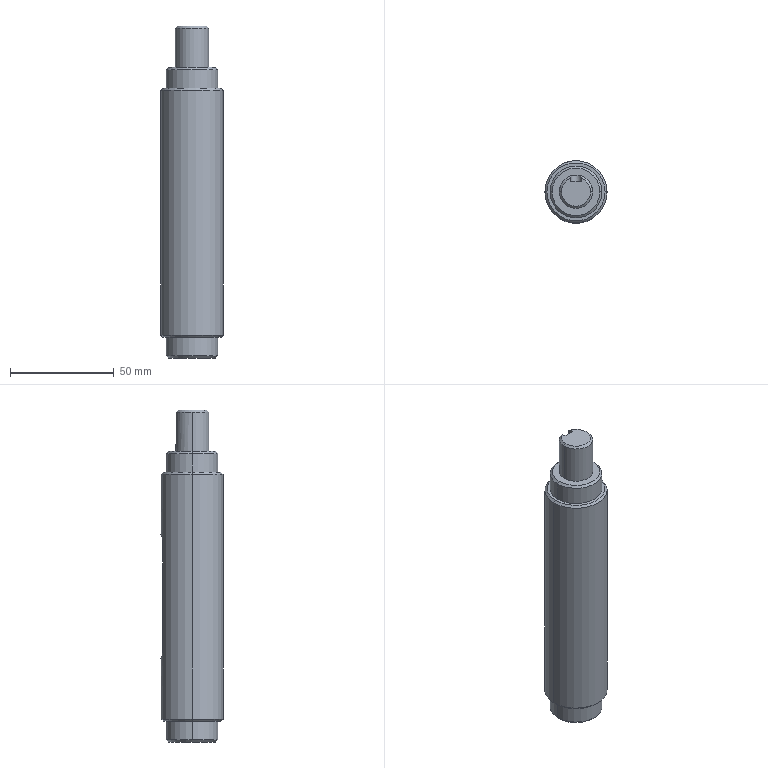Component | SolidWorks | WT-FLD-EJG-1212-00-008-1 | 1 solid | 33 faces | box 30 x 30 x 160 mm | volume 95493 mm3 | cone 11 | cylinder 11 | plane 11 | commonest cylinder face diameters 25 x4 30 x2 16 x2 10 x2 5 x1 | material AISI 1045 Steel, cold drawn
build123d program:
from build123d import *

# Parameters (mm, degrees)
CUT_EXTRUDE1_START  = 10
CUT_EXTRUDE1_DEPTH  = 64.144
SKETCH3_R           = 8
BOSS_EXTRUDE1_DEPTH = 20
CHAMFER1_SIZE       = 1
CUT_EXTRUDE2_START  = 5
CUT_EXTRUDE2_DEPTH  = 88.466


with BuildPart() as part:
    # Sketch1 → Revolve1 (revolve)
    with BuildSketch(Plane.XY, mode=Mode.PRIVATE) as revolve1_sk:
        Polygon((-70, 12.5), (-60, 12.5), (-60, 15), (60, 15), (60, 12.5), (70, 12.5), (70, 0), (-70, 0), align=None)
    revolve(revolve1_sk.sketch.rotate(Axis((-70, 0, 0), (1, 0, 0)), 90), axis=Axis((-70, 0, 0), (1, 0, 0)))

    # Sketch2 → Cut-Extrude1 (cut, through all)
    with BuildSketch(Plane(origin=(0, 0, 0), x_dir=(1, 0, 0), z_dir=(0, 1, 0)).offset(CUT_EXTRUDE1_START)):
        with BuildLine():
            Line((-25, 5), (25, 5))
            ThreePointArc((25, 5), (30, 0), (25, -5))
            Line((25, -5), (-25, -5))
            ThreePointArc((-25, -5), (-30, 0), (-25, 5))
        make_face()
    extrude(amount=CUT_EXTRUDE1_DEPTH, mode=Mode.SUBTRACT)

    # Sketch3 → Boss-Extrude1 (add)
    with BuildSketch(Plane(origin=(70, 0, 0), x_dir=(0, 0, -1), z_dir=(1, 0, 0))):
        with Locations(Location((0, 0, 0), (0, 0, 180))):
            Circle(SKETCH3_R)
    extrude(amount=BOSS_EXTRUDE1_DEPTH)

    # Chamfer1
    chamfer1_edges = [part.edges().sort_by_distance(p)[0] for p in [
        (90, 0, -8),
        (-70, 0, -12.5),
        (-60, 0, -15),
        (60, 0, -15),
        (70, 0, -12.5),
    ]]
    chamfer(chamfer1_edges, length=CHAMFER1_SIZE)

    # Sketch4 → Cut-Extrude2 (cut, through all)
    with BuildSketch(Plane(origin=(0, 0, 0), x_dir=(1, 0, 0), z_dir=(0, 1, 0)).offset(CUT_EXTRUDE2_START)):
        with BuildLine():
            Line((75, 2.5), (95, 2.5))
            ThreePointArc((95, 2.5), (97.5, 0), (95, -2.5))
            Line((95, -2.5), (75, -2.5))
            ThreePointArc((75, -2.5), (72.5, 0), (75, 2.5))
        make_face()
    extrude(amount=CUT_EXTRUDE2_DEPTH, mode=Mode.SUBTRACT)


solid = part.part

# Placed as in the assembly
solid = solid.moved(Location((0, 0, 0), (0, -90, 0)))
STEP:
#1=COLOUR_RGB('',0.7922,0.8196,0.9333);
#2=FILL_AREA_STYLE_COLOUR('',#1);
#3=FILL_AREA_STYLE('',(#2));
#4=SURFACE_STYLE_FILL_AREA(#3);
#5=SURFACE_SIDE_STYLE('',(#4));
#6=SURFACE_STYLE_USAGE(.BOTH.,#5);
#7=PRESENTATION_STYLE_ASSIGNMENT((#6));
#8=CARTESIAN_POINT('',(-0.5512,0.,-2.362));
#9=VERTEX_POINT('',#8);
#10=CARTESIAN_POINT('',(0.5512,0.,-2.362));
#11=VERTEX_POINT('',#10);
#12=CARTESIAN_POINT('',(0.,0.,-2.362));
#13=DIRECTION('',(0.,0.,-1.));
#14=DIRECTION('',(1.,0.,0.));
#15=AXIS2_PLACEMENT_3D('',#12,#13,#14);
#16=CIRCLE('',#15,0.5512);
#17=EDGE_CURVE('',#9,#11,#16,.T.);
#18=ORIENTED_EDGE('',*,*,#17,.F.);
#19=CARTESIAN_POINT('',(-0.5906,-0.,-2.323));
#20=VERTEX_POINT('',#19);
#21=CARTESIAN_POINT('',(-0.5512,0.,-2.362));
#22=DIRECTION('',(-0.7071,0.,0.7071));
#23=VECTOR('',#22,39.37);
#24=LINE('',#21,#23);
#25=EDGE_CURVE('',#9,#20,#24,.T.);
#26=ORIENTED_EDGE('',*,*,#25,.T.);
#27=CARTESIAN_POINT('',(0.5906,0.,-2.323));
#28=VERTEX_POINT('',#27);
#29=CARTESIAN_POINT('',(0.,0.,-2.323));
#30=DIRECTION('',(0.,0.,1.));
#31=DIRECTION('',(1.,0.,0.));
#32=AXIS2_PLACEMENT_3D('',#29,#30,#31);
#33=CIRCLE('',#32,0.5906);
#34=EDGE_CURVE('',#28,#20,#33,.T.);
#35=ORIENTED_EDGE('',*,*,#34,.F.);
#36=CARTESIAN_POINT('',(0.5512,0.,-2.362));
#37=DIRECTION('',(0.7071,0.,0.7071));
#38=VECTOR('',#37,39.37);
#39=LINE('',#36,#38);
#40=EDGE_CURVE('',#11,#28,#39,.T.);
#41=ORIENTED_EDGE('',*,*,#40,.F.);
#42=EDGE_LOOP('',(#18,#26,#35,#41));
#43=FACE_OUTER_BOUND('',#42,.T.);
#44=CARTESIAN_POINT('',(0.,0.,-2.362));
#45=DIRECTION('',(0.,0.,1.));
#46=DIRECTION('',(1.,0.,0.));
#47=AXIS2_PLACEMENT_3D('',#44,#45,#46);
#48=CONICAL_SURFACE('',#47,0.5512,0.7854);
#49=ADVANCED_FACE('',(#43),#48,.T.);
#50=CARTESIAN_POINT('',(-0.4528,0.,-2.756));
#51=VERTEX_POINT('',#50);
#52=CARTESIAN_POINT('',(0.4528,0.,-2.756));
#53=VERTEX_POINT('',#52);
#54=CARTESIAN_POINT('',(0.,0.,-2.756));
#55=DIRECTION('',(0.,0.,-1.));
#56=DIRECTION('',(1.,0.,0.));
#57=AXIS2_PLACEMENT_3D('',#54,#55,#56);
#58=CIRCLE('',#57,0.4528);
#59=EDGE_CURVE('',#51,#53,#58,.T.);
#60=ORIENTED_EDGE('',*,*,#59,.F.);
#61=CARTESIAN_POINT('',(-0.4921,-0.,-2.717));
#62=VERTEX_POINT('',#61);
#63=CARTESIAN_POINT('',(-0.4528,0.,-2.756));
#64=DIRECTION('',(-0.7071,0.,0.7071));
#65=VECTOR('',#64,39.37);
#66=LINE('',#63,#65);
#67=EDGE_CURVE('',#51,#62,#66,.T.);
#68=ORIENTED_EDGE('',*,*,#67,.T.);
#69=CARTESIAN_POINT('',(0.4921,0.,-2.717));
#70=VERTEX_POINT('',#69);
#71=CARTESIAN_POINT('',(0.,0.,-2.717));
#72=DIRECTION('',(0.,0.,1.));
#73=DIRECTION('',(1.,0.,0.));
#74=AXIS2_PLACEMENT_3D('',#71,#72,#73);
#75=CIRCLE('',#74,0.4921);
#76=EDGE_CURVE('',#70,#62,#75,.T.);
#77=ORIENTED_EDGE('',*,*,#76,.F.);
#78=CARTESIAN_POINT('',(0.4528,0.,-2.756));
#79=DIRECTION('',(0.7071,0.,0.7071));
#80=VECTOR('',#79,39.37);
#81=LINE('',#78,#80);
#82=EDGE_CURVE('',#53,#70,#81,.T.);
#83=ORIENTED_EDGE('',*,*,#82,.F.);
#84=EDGE_LOOP('',(#60,#68,#77,#83));
#85=FACE_OUTER_BOUND('',#84,.T.);
#86=CARTESIAN_POINT('',(0.,0.,-2.756));
#87=DIRECTION('',(0.,0.,1.));
#88=DIRECTION('',(1.,0.,0.));
#89=AXIS2_PLACEMENT_3D('',#86,#87,#88);
#90=CONICAL_SURFACE('',#89,0.4528,0.7854);
#91=ADVANCED_FACE('',(#85),#90,.T.);
#92=CARTESIAN_POINT('',(0.5512,0.,2.362));
#93=VERTEX_POINT('',#92);
#94=CARTESIAN_POINT('',(-0.5512,-0.,2.362));
#95=VERTEX_POINT('',#94);
#96=CARTESIAN_POINT('',(0.,0.,2.362));
#97=DIRECTION('',(0.,0.,1.));
#98=DIRECTION('',(-1.,-0.,0.));
#99=AXIS2_PLACEMENT_3D('',#96,#97,#98);
#100=CIRCLE('',#99,0.5512);
#101=EDGE_CURVE('',#93,#95,#100,.T.);
#102=ORIENTED_EDGE('',*,*,#101,.F.);
#103=CARTESIAN_POINT('',(0.5906,0.,2.323));
#104=VERTEX_POINT('',#103);
#105=CARTESIAN_POINT('',(0.5906,0.,2.323));
#106=DIRECTION('',(0.7071,0.,-0.7071));
#107=VECTOR('',#106,39.37);
#108=LINE('',#105,#107);
#109=EDGE_CURVE('',#93,#104,#108,.T.);
#110=ORIENTED_EDGE('',*,*,#109,.T.);
#111=CARTESIAN_POINT('',(-0.5906,-0.,2.323));
#112=VERTEX_POINT('',#111);
#113=CARTESIAN_POINT('',(0.,0.,2.323));
#114=DIRECTION('',(0.,0.,-1.));
#115=DIRECTION('',(-1.,-0.,0.));
#116=AXIS2_PLACEMENT_3D('',#113,#114,#115);
#117=CIRCLE('',#116,0.5906);
#118=EDGE_CURVE('',#112,#104,#117,.T.);
#119=ORIENTED_EDGE('',*,*,#118,.F.);
#120=CARTESIAN_POINT('',(-0.5906,-0.,2.323));
#121=DIRECTION('',(-0.7071,-0.,-0.7071));
#122=VECTOR('',#121,39.37);
#123=LINE('',#120,#122);
#124=EDGE_CURVE('',#95,#112,#123,.T.);
#125=ORIENTED_EDGE('',*,*,#124,.F.);
#126=EDGE_LOOP('',(#102,#110,#119,#125));
#127=FACE_OUTER_BOUND('',#126,.T.);
#128=CARTESIAN_POINT('',(0.,0.,2.323));
#129=DIRECTION('',(0.,0.,-1.));
#130=DIRECTION('',(-1.,-0.,0.));
#131=AXIS2_PLACEMENT_3D('',#128,#129,#130);
#132=CONICAL_SURFACE('',#131,0.5906,0.7854);
#133=ADVANCED_FACE('',(#127),#132,.T.);
#134=CARTESIAN_POINT('',(0.4528,0.,2.756));
#135=VERTEX_POINT('',#134);
#136=CARTESIAN_POINT('',(-0.4528,-0.,2.756));
#137=VERTEX_POINT('',#136);
#138=CARTESIAN_POINT('',(0.,0.,2.756));
#139=DIRECTION('',(0.,0.,1.));
#140=DIRECTION('',(-1.,-0.,0.));
#141=AXIS2_PLACEMENT_3D('',#138,#139,#140);
#142=CIRCLE('',#141,0.4528);
#143=EDGE_CURVE('',#135,#137,#142,.T.);
#144=ORIENTED_EDGE('',*,*,#143,.F.);
#145=CARTESIAN_POINT('',(0.4921,0.,2.717));
#146=VERTEX_POINT('',#145);
#147=CARTESIAN_POINT('',(0.4921,0.,2.717));
#148=DIRECTION('',(0.7071,0.,-0.7071));
#149=VECTOR('',#148,39.37);
#150=LINE('',#147,#149);
#151=EDGE_CURVE('',#135,#146,#150,.T.);
#152=ORIENTED_EDGE('',*,*,#151,.T.);
#153=CARTESIAN_POINT('',(-0.4921,-0.,2.717));
#154=VERTEX_POINT('',#153);
#155=CARTESIAN_POINT('',(0.,0.,2.717));
#156=DIRECTION('',(0.,0.,-1.));
#157=DIRECTION('',(-1.,-0.,0.));
#158=AXIS2_PLACEMENT_3D('',#155,#156,#157);
#159=CIRCLE('',#158,0.4921);
#160=EDGE_CURVE('',#154,#146,#159,.T.);
#161=ORIENTED_EDGE('',*,*,#160,.F.);
#162=CARTESIAN_POINT('',(-0.4921,-0.,2.717));
#163=DIRECTION('',(-0.7071,-0.,-0.7071));
#164=VECTOR('',#163,39.37);
#165=LINE('',#162,#164);
#166=EDGE_CURVE('',#137,#154,#165,.T.);
#167=ORIENTED_EDGE('',*,*,#166,.F.);
#168=EDGE_LOOP('',(#144,#152,#161,#167));
#169=FACE_OUTER_BOUND('',#168,.T.);
#170=CARTESIAN_POINT('',(0.,0.,2.717));
#171=DIRECTION('',(0.,0.,-1.));
#172=DIRECTION('',(-1.,-0.,0.));
#173=AXIS2_PLACEMENT_3D('',#170,#171,#172);
#174=CONICAL_SURFACE('',#173,0.4921,0.7854);
#175=ADVANCED_FACE('',(#169),#174,.T.);
#176=CARTESIAN_POINT('',(-0.4921,-0.,-2.362));
#177=VERTEX_POINT('',#176);
#178=CARTESIAN_POINT('',(0.4921,0.,-2.362));
#179=VERTEX_POINT('',#178);
#180=CARTESIAN_POINT('',(0.,0.,-2.362));
#181=DIRECTION('',(0.,0.,-1.));
#182=DIRECTION('',(-1.,-0.,0.));
#183=AXIS2_PLACEMENT_3D('',#180,#181,#182);
#184=CIRCLE('',#183,0.4921);
#185=EDGE_CURVE('',#177,#179,#184,.T.);
#186=ORIENTED_EDGE('',*,*,#185,.T.);
#187=CARTESIAN_POINT('',(0.4921,0.,-2.756));
#188=DIRECTION('',(0.,0.,-1.));
#189=VECTOR('',#188,39.37);
#190=LINE('',#187,#189);
#191=EDGE_CURVE('',#179,#70,#190,.T.);
#192=ORIENTED_EDGE('',*,*,#191,.T.);
#193=ORIENTED_EDGE('',*,*,#76,.T.);
#194=CARTESIAN_POINT('',(-0.4921,-0.,-2.756));
#195=DIRECTION('',(0.,0.,-1.));
#196=VECTOR('',#195,39.37);
#197=LINE('',#194,#196);
#198=EDGE_CURVE('',#177,#62,#197,.T.);
#199=ORIENTED_EDGE('',*,*,#198,.F.);
#200=EDGE_LOOP('',(#186,#192,#193,#199));
#201=FACE_OUTER_BOUND('',#200,.T.);
#202=CARTESIAN_POINT('',(0.,0.,-2.756));
#203=DIRECTION('',(0.,0.,-1.));
#204=DIRECTION('',(-1.,-0.,0.));
#205=AXIS2_PLACEMENT_3D('',#202,#203,#204);
#206=CYLINDRICAL_SURFACE('',#205,0.4921);
#207=ADVANCED_FACE('',(#201),#206,.T.);
#208=ORIENTED_EDGE('',*,*,#160,.T.);
#209=CARTESIAN_POINT('',(0.4921,0.,2.362));
#210=VERTEX_POINT('',#209);
#211=CARTESIAN_POINT('',(0.4921,0.,-2.756));
#212=DIRECTION('',(0.,0.,-1.));
#213=VECTOR('',#212,39.37);
#214=LINE('',#211,#213);
#215=EDGE_CURVE('',#146,#210,#214,.T.);
#216=ORIENTED_EDGE('',*,*,#215,.T.);
#217=CARTESIAN_POINT('',(-0.4921,-0.,2.362));
#218=VERTEX_POINT('',#217);
#219=CARTESIAN_POINT('',(0.,0.,2.362));
#220=DIRECTION('',(0.,0.,-1.));
#221=DIRECTION('',(-1.,-0.,0.));
#222=AXIS2_PLACEMENT_3D('',#219,#220,#221);
#223=CIRCLE('',#222,0.4921);
#224=EDGE_CURVE('',#218,#210,#223,.T.);
#225=ORIENTED_EDGE('',*,*,#224,.F.);
#226=CARTESIAN_POINT('',(-0.4921,-0.,-2.756));
#227=DIRECTION('',(0.,0.,-1.));
#228=VECTOR('',#227,39.37);
#229=LINE('',#226,#228);
#230=EDGE_CURVE('',#154,#218,#229,.T.);
#231=ORIENTED_EDGE('',*,*,#230,.F.);
#232=EDGE_LOOP('',(#208,#216,#225,#231));
#233=FACE_OUTER_BOUND('',#232,.T.);
#234=CARTESIAN_POINT('',(0.,0.,-2.756));
#235=DIRECTION('',(0.,0.,-1.));
#236=DIRECTION('',(-1.,-0.,0.));
#237=AXIS2_PLACEMENT_3D('',#234,#235,#236);
#238=CYLINDRICAL_SURFACE('',#237,0.4921);
#239=ADVANCED_FACE('',(#233),#238,.T.);
#240=CARTESIAN_POINT('',(-0.1969,0.5568,0.9843));
#241=VERTEX_POINT('',#240);
#242=CARTESIAN_POINT('',(0.1969,0.5568,0.9843));
#243=VERTEX_POINT('',#242);
#244=CARTESIAN_POINT('',(-0.1969,0.5568,0.9843));
#245=CARTESIAN_POINT('',(-0.1969,0.5568,0.9974));
#246=CARTESIAN_POINT('',(-0.1956,0.5572,1.01));
#247=CARTESIAN_POINT('',(-0.1905,0.559,1.035));
#248=CARTESIAN_POINT('',(-0.1867,0.5603,1.048));
#249=CARTESIAN_POINT('',(-0.1768,0.5635,1.072));
#250=CARTESIAN_POINT('',(-0.1707,0.5654,1.083));
#251=CARTESIAN_POINT('',(-0.1565,0.5695,1.104));
#252=CARTESIAN_POINT('',(-0.1482,0.5717,1.114));
#253=CARTESIAN_POINT('',(-0.1302,0.5761,1.132));
#254=CARTESIAN_POINT('',(-0.1204,0.5783,1.141));
#255=CARTESIAN_POINT('',(-0.09888,0.5823,1.155));
#256=CARTESIAN_POINT('',(-0.08758,0.5841,1.161));
#257=CARTESIAN_POINT('',(-0.06985,0.5864,1.168));
#258=CARTESIAN_POINT('',(-0.0638,0.5871,1.171));
#259=CARTESIAN_POINT('',(-0.05143,0.5883,1.174));
#260=CARTESIAN_POINT('',(-0.04507,0.5889,1.176));
#261=CARTESIAN_POINT('',(-0.02599,0.5901,1.18));
#262=CARTESIAN_POINT('',(-0.01315,0.5905,1.181));
#263=CARTESIAN_POINT('',(0.01273,0.5906,1.181));
#264=CARTESIAN_POINT('',(0.02588,0.5901,1.18));
#265=CARTESIAN_POINT('',(0.05121,0.5885,1.175));
#266=CARTESIAN_POINT('',(0.06353,0.5872,1.171));
#267=CARTESIAN_POINT('',(0.08749,0.5842,1.161));
#268=CARTESIAN_POINT('',(0.09885,0.5823,1.155));
#269=CARTESIAN_POINT('',(0.1201,0.5783,1.141));
#270=CARTESIAN_POINT('',(0.1301,0.5761,1.133));
#271=CARTESIAN_POINT('',(0.1482,0.5717,1.114));
#272=CARTESIAN_POINT('',(0.1563,0.5695,1.105));
#273=CARTESIAN_POINT('',(0.1706,0.5654,1.083));
#274=CARTESIAN_POINT('',(0.1768,0.5635,1.072));
#275=CARTESIAN_POINT('',(0.1866,0.5603,1.048));
#276=CARTESIAN_POINT('',(0.1904,0.559,1.036));
#277=CARTESIAN_POINT('',(0.1955,0.5572,1.01));
#278=CARTESIAN_POINT('',(0.1969,0.5568,0.9974));
#279=CARTESIAN_POINT('',(0.1969,0.5568,0.9843));
#280=B_SPLINE_CURVE_WITH_KNOTS('',3,(#244,#245,#246,#247,#248,#249,#250,#251,#252,#253,#254,#255,#256,#257,#258,#259,#260,#261,#262,#263,#264,#265,#266,#267,#268,#269,#270,#271,#272,#273,#274,#275,#276,#277,#278,#279),.UNSPECIFIED.,.F.,.F.,(4,2,2,2,2,2,2,2,2,2,2,2,2,2,2,2,2,4),(0.,0.0009837,0.001967,0.002951,0.003935,0.004919,0.005902,0.006394,0.006886,0.00787,0.008853,0.009837,0.01082,0.0118,0.01279,0.01377,0.01476,0.01574),.UNSPECIFIED.);
#281=EDGE_CURVE('',#241,#243,#280,.T.);
#282=ORIENTED_EDGE('',*,*,#281,.F.);
#283=CARTESIAN_POINT('',(-0.1969,0.5568,-0.9843));
#284=VERTEX_POINT('',#283);
#285=CARTESIAN_POINT('',(-0.1969,0.5568,-2.756));
#286=DIRECTION('',(0.,0.,1.));
#287=VECTOR('',#286,39.37);
#288=LINE('',#285,#287);
#289=EDGE_CURVE('',#284,#241,#288,.T.);
#290=ORIENTED_EDGE('',*,*,#289,.F.);
#291=CARTESIAN_POINT('',(0.1969,0.5568,-0.9843));
#292=VERTEX_POINT('',#291);
#293=CARTESIAN_POINT('',(0.1969,0.5568,-0.9843));
#294=CARTESIAN_POINT('',(0.1969,0.5568,-0.9974));
#295=CARTESIAN_POINT('',(0.1956,0.5572,-1.01));
#296=CARTESIAN_POINT('',(0.1905,0.559,-1.035));
#297=CARTESIAN_POINT('',(0.1867,0.5603,-1.048));
#298=CARTESIAN_POINT('',(0.1768,0.5635,-1.072));
#299=CARTESIAN_POINT('',(0.1707,0.5654,-1.083));
#300=CARTESIAN_POINT('',(0.1565,0.5695,-1.104));
#301=CARTESIAN_POINT('',(0.1482,0.5717,-1.114));
#302=CARTESIAN_POINT('',(0.1302,0.5761,-1.132));
#303=CARTESIAN_POINT('',(0.1204,0.5783,-1.141));
#304=CARTESIAN_POINT('',(0.09888,0.5823,-1.155));
#305=CARTESIAN_POINT('',(0.08758,0.5841,-1.161));
#306=CARTESIAN_POINT('',(0.06985,0.5864,-1.168));
#307=CARTESIAN_POINT('',(0.0638,0.5871,-1.171));
#308=CARTESIAN_POINT('',(0.05143,0.5883,-1.174));
#309=CARTESIAN_POINT('',(0.04507,0.5889,-1.176));
#310=CARTESIAN_POINT('',(0.02599,0.5901,-1.18));
#311=CARTESIAN_POINT('',(0.01315,0.5905,-1.181));
#312=CARTESIAN_POINT('',(-0.01273,0.5906,-1.181));
#313=CARTESIAN_POINT('',(-0.02588,0.5901,-1.18));
#314=CARTESIAN_POINT('',(-0.05121,0.5885,-1.175));
#315=CARTESIAN_POINT('',(-0.06353,0.5872,-1.171));
#316=CARTESIAN_POINT('',(-0.08749,0.5842,-1.161));
#317=CARTESIAN_POINT('',(-0.09885,0.5823,-1.155));
#318=CARTESIAN_POINT('',(-0.1201,0.5783,-1.141));
#319=CARTESIAN_POINT('',(-0.1301,0.5761,-1.133));
#320=CARTESIAN_POINT('',(-0.1482,0.5717,-1.114));
#321=CARTESIAN_POINT('',(-0.1563,0.5695,-1.105));
#322=CARTESIAN_POINT('',(-0.1706,0.5654,-1.083));
#323=CARTESIAN_POINT('',(-0.1768,0.5635,-1.072));
#324=CARTESIAN_POINT('',(-0.1866,0.5603,-1.048));
#325=CARTESIAN_POINT('',(-0.1904,0.559,-1.036));
#326=CARTESIAN_POINT('',(-0.1955,0.5572,-1.01));
#327=CARTESIAN_POINT('',(-0.1969,0.5568,-0.9974));
#328=CARTESIAN_POINT('',(-0.1969,0.5568,-0.9843));
#329=B_SPLINE_CURVE_WITH_KNOTS('',3,(#293,#294,#295,#296,#297,#298,#299,#300,#301,#302,#303,#304,#305,#306,#307,#308,#309,#310,#311,#312,#313,#314,#315,#316,#317,#318,#319,#320,#321,#322,#323,#324,#325,#326,#327,#328),.UNSPECIFIED.,.F.,.F.,(4,2,2,2,2,2,2,2,2,2,2,2,2,2,2,2,2,4),(0.,0.0009837,0.001967,0.002951,0.003935,0.004919,0.005902,0.006394,0.006886,0.00787,0.008853,0.009837,0.01082,0.0118,0.01279,0.01377,0.01476,0.01574),.UNSPECIFIED.);
#330=EDGE_CURVE('',#292,#284,#329,.T.);
#331=ORIENTED_EDGE('',*,*,#330,.F.);
#332=CARTESIAN_POINT('',(0.1969,0.5568,-2.756));
#333=DIRECTION('',(0.,0.,-1.));
#334=VECTOR('',#333,39.37);
#335=LINE('',#332,#334);
#336=EDGE_CURVE('',#243,#292,#335,.T.);
#337=ORIENTED_EDGE('',*,*,#336,.F.);
#338=EDGE_LOOP('',(#282,#290,#331,#337));
#339=FACE_BOUND('',#338,.T.);
#340=ORIENTED_EDGE('',*,*,#118,.T.);
#341=CARTESIAN_POINT('',(0.5906,0.,-2.756));
#342=DIRECTION('',(0.,0.,-1.));
#343=VECTOR('',#342,39.37);
#344=LINE('',#341,#343);
#345=EDGE_CURVE('',#104,#28,#344,.T.);
#346=ORIENTED_EDGE('',*,*,#345,.T.);
#347=ORIENTED_EDGE('',*,*,#34,.T.);
#348=CARTESIAN_POINT('',(-0.5906,-0.,-2.756));
#349=DIRECTION('',(0.,0.,-1.));
#350=VECTOR('',#349,39.37);
#351=LINE('',#348,#350);
#352=EDGE_CURVE('',#112,#20,#351,.T.);
#353=ORIENTED_EDGE('',*,*,#352,.F.);
#354=EDGE_LOOP('',(#340,#346,#347,#353));
#355=FACE_OUTER_BOUND('',#354,.T.);
#356=CARTESIAN_POINT('',(0.,0.,-2.756));
#357=DIRECTION('',(0.,0.,-1.));
#358=DIRECTION('',(-1.,-0.,0.));
#359=AXIS2_PLACEMENT_3D('',#356,#357,#358);
#360=CYLINDRICAL_SURFACE('',#359,0.5906);
#361=ADVANCED_FACE('',(#339,#355),#360,.T.);
#362=CARTESIAN_POINT('',(0.2756,0.,3.543));
#363=VERTEX_POINT('',#362);
#364=CARTESIAN_POINT('',(0.09843,0.2574,3.543));
#365=VERTEX_POINT('',#364);
#366=CARTESIAN_POINT('',(0.,0.,3.543));
#367=DIRECTION('',(0.,0.,1.));
#368=DIRECTION('',(1.,0.,0.));
#369=AXIS2_PLACEMENT_3D('',#366,#367,#368);
#370=CIRCLE('',#369,0.2756);
#371=EDGE_CURVE('',#363,#365,#370,.T.);
#372=ORIENTED_EDGE('',*,*,#371,.F.);
#373=CARTESIAN_POINT('',(0.315,0.,3.504));
#374=VERTEX_POINT('',#373);
#375=CARTESIAN_POINT('',(0.2756,0.,3.543));
#376=DIRECTION('',(0.7071,0.,-0.7071));
#377=VECTOR('',#376,39.37);
#378=LINE('',#375,#377);
#379=EDGE_CURVE('',#363,#374,#378,.T.);
#380=ORIENTED_EDGE('',*,*,#379,.T.);
#381=CARTESIAN_POINT('',(0.09843,0.2992,3.504));
#382=VERTEX_POINT('',#381);
#383=CARTESIAN_POINT('',(0.,0.,3.504));
#384=DIRECTION('',(0.,0.,-1.));
#385=DIRECTION('',(1.,-0.,0.));
#386=AXIS2_PLACEMENT_3D('',#383,#384,#385);
#387=CIRCLE('',#386,0.315);
#388=EDGE_CURVE('',#382,#374,#387,.T.);
#389=ORIENTED_EDGE('',*,*,#388,.F.);
#390=CARTESIAN_POINT('',(0.09843,0.2992,3.504));
#391=CARTESIAN_POINT('',(0.09843,0.2853,3.517));
#392=CARTESIAN_POINT('',(0.09843,0.2714,3.53));
#393=CARTESIAN_POINT('',(0.09843,0.2574,3.543));
#394=B_SPLINE_CURVE_WITH_KNOTS('',3,(#390,#391,#392,#393),.UNSPECIFIED.,.F.,.F.,(4,4),(0.005308,0.006766),.UNSPECIFIED.);
#395=EDGE_CURVE('',#382,#365,#394,.T.);
#396=ORIENTED_EDGE('',*,*,#395,.T.);
#397=EDGE_LOOP('',(#372,#380,#389,#396));
#398=FACE_OUTER_BOUND('',#397,.T.);
#399=CARTESIAN_POINT('',(0.,0.,3.543));
#400=DIRECTION('',(0.,0.,-1.));
#401=DIRECTION('',(-1.,-0.,0.));
#402=AXIS2_PLACEMENT_3D('',#399,#400,#401);
#403=CONICAL_SURFACE('',#402,0.2756,0.7854);
#404=ADVANCED_FACE('',(#398),#403,.T.);
#405=ORIENTED_EDGE('',*,*,#379,.F.);
#406=CARTESIAN_POINT('',(-0.2756,-0.,3.543));
#407=VERTEX_POINT('',#406);
#408=CARTESIAN_POINT('',(0.,0.,3.543));
#409=DIRECTION('',(0.,0.,1.));
#410=DIRECTION('',(1.,0.,0.));
#411=AXIS2_PLACEMENT_3D('',#408,#409,#410);
#412=CIRCLE('',#411,0.2756);
#413=EDGE_CURVE('',#407,#363,#412,.T.);
#414=ORIENTED_EDGE('',*,*,#413,.F.);
#415=CARTESIAN_POINT('',(-0.315,-0.,3.504));
#416=VERTEX_POINT('',#415);
#417=CARTESIAN_POINT('',(-0.2756,-0.,3.543));
#418=DIRECTION('',(-0.7071,-0.,-0.7071));
#419=VECTOR('',#418,39.37);
#420=LINE('',#417,#419);
#421=EDGE_CURVE('',#407,#416,#420,.T.);
#422=ORIENTED_EDGE('',*,*,#421,.T.);
#423=CARTESIAN_POINT('',(0.,0.,3.504));
#424=DIRECTION('',(0.,0.,-1.));
#425=DIRECTION('',(1.,0.,0.));
#426=AXIS2_PLACEMENT_3D('',#423,#424,#425);
#427=CIRCLE('',#426,0.315);
#428=EDGE_CURVE('',#374,#416,#427,.T.);
#429=ORIENTED_EDGE('',*,*,#428,.F.);
#430=EDGE_LOOP('',(#405,#414,#422,#429));
#431=FACE_OUTER_BOUND('',#430,.T.);
#432=CARTESIAN_POINT('',(0.,0.,3.543));
#433=DIRECTION('',(0.,0.,-1.));
#434=DIRECTION('',(-1.,-0.,0.));
#435=AXIS2_PLACEMENT_3D('',#432,#433,#434);
#436=CONICAL_SURFACE('',#435,0.2756,0.7854);
#437=ADVANCED_FACE('',(#431),#436,.T.);
#438=ORIENTED_EDGE('',*,*,#388,.T.);
#439=CARTESIAN_POINT('',(0.315,0.,2.756));
#440=VERTEX_POINT('',#439);
#441=CARTESIAN_POINT('',(0.315,0.,3.543));
#442=DIRECTION('',(0.,0.,-1.));
#443=VECTOR('',#442,39.37);
#444=LINE('',#441,#443);
#445=EDGE_CURVE('',#374,#440,#444,.T.);
#446=ORIENTED_EDGE('',*,*,#445,.T.);
#447=CARTESIAN_POINT('',(-0.315,-0.,2.756));
#448=VERTEX_POINT('',#447);
#449=CARTESIAN_POINT('',(0.,0.,2.756));
#450=DIRECTION('',(0.,0.,1.));
#451=DIRECTION('',(-1.,-0.,0.));
#452=AXIS2_PLACEMENT_3D('',#449,#450,#451);
#453=CIRCLE('',#452,0.315);
#454=EDGE_CURVE('',#440,#448,#453,.T.);
#455=ORIENTED_EDGE('',*,*,#454,.T.);
#456=CARTESIAN_POINT('',(-0.315,-0.,3.543));
#457=DIRECTION('',(0.,0.,-1.));
#458=VECTOR('',#457,39.37);
#459=LINE('',#456,#458);
#460=EDGE_CURVE('',#416,#448,#459,.T.);
#461=ORIENTED_EDGE('',*,*,#460,.F.);
#462=CARTESIAN_POINT('',(-0.09843,0.2992,3.504));
#463=VERTEX_POINT('',#462);
#464=CARTESIAN_POINT('',(0.,0.,3.504));
#465=DIRECTION('',(0.,0.,-1.));
#466=DIRECTION('',(1.,0.,0.));
#467=AXIS2_PLACEMENT_3D('',#464,#465,#466);
#468=CIRCLE('',#467,0.315);
#469=EDGE_CURVE('',#416,#463,#468,.T.);
#470=ORIENTED_EDGE('',*,*,#469,.T.);
#471=CARTESIAN_POINT('',(-0.09843,0.2992,2.953));
#472=VERTEX_POINT('',#471);
#473=CARTESIAN_POINT('',(-0.09843,0.2992,3.543));
#474=DIRECTION('',(0.,0.,1.));
#475=VECTOR('',#474,39.37);
#476=LINE('',#473,#475);
#477=EDGE_CURVE('',#472,#463,#476,.T.);
#478=ORIENTED_EDGE('',*,*,#477,.F.);
#479=CARTESIAN_POINT('',(0.09843,0.2992,2.953));
#480=VERTEX_POINT('',#479);
#481=CARTESIAN_POINT('',(0.09843,0.2992,2.953));
#482=CARTESIAN_POINT('',(0.09843,0.2992,2.946));
#483=CARTESIAN_POINT('',(0.09778,0.2994,2.94));
#484=CARTESIAN_POINT('',(0.09525,0.3002,2.927));
#485=CARTESIAN_POINT('',(0.09334,0.3008,2.921));
#486=CARTESIAN_POINT('',(0.08839,0.3023,2.909));
#487=CARTESIAN_POINT('',(0.08537,0.3032,2.903));
#488=CARTESIAN_POINT('',(0.07823,0.3051,2.893));
#489=CARTESIAN_POINT('',(0.07411,0.3062,2.888));
#490=CARTESIAN_POINT('',(0.06059,0.3092,2.874));
#491=CARTESIAN_POINT('',(0.04968,0.3112,2.867));
#492=CARTESIAN_POINT('',(0.03194,0.3134,2.859));
#493=CARTESIAN_POINT('',(0.0257,0.314,2.858));
#494=CARTESIAN_POINT('',(0.01298,0.3148,2.855));
#495=CARTESIAN_POINT('',(0.006564,0.315,2.854));
#496=CARTESIAN_POINT('',(-0.006364,0.315,2.854));
#497=CARTESIAN_POINT('',(-0.01293,0.3148,2.855));
#498=CARTESIAN_POINT('',(-0.02559,0.314,2.857));
#499=CARTESIAN_POINT('',(-0.03175,0.3134,2.859));
#500=CARTESIAN_POINT('',(-0.04372,0.312,2.864));
#501=CARTESIAN_POINT('',(-0.04941,0.3111,2.867));
#502=CARTESIAN_POINT('',(-0.06003,0.3092,2.874));
#503=CARTESIAN_POINT('',(-0.06504,0.3082,2.879));
#504=CARTESIAN_POINT('',(-0.07412,0.3062,2.888));
#505=CARTESIAN_POINT('',(-0.07816,0.3051,2.893));
#506=CARTESIAN_POINT('',(-0.08529,0.3032,2.903));
#507=CARTESIAN_POINT('',(-0.08838,0.3023,2.909));
#508=CARTESIAN_POINT('',(-0.09332,0.3008,2.921));
#509=CARTESIAN_POINT('',(-0.0952,0.3002,2.927));
#510=CARTESIAN_POINT('',(-0.09777,0.2994,2.94));
#511=CARTESIAN_POINT('',(-0.09843,0.2992,2.946));
#512=CARTESIAN_POINT('',(-0.09843,0.2992,2.953));
#513=B_SPLINE_CURVE_WITH_KNOTS('',3,(#481,#482,#483,#484,#485,#486,#487,#488,#489,#490,#491,#492,#493,#494,#495,#496,#497,#498,#499,#500,#501,#502,#503,#504,#505,#506,#507,#508,#509,#510,#511,#512),.UNSPECIFIED.,.F.,.F.,(4,2,2,2,2,2,2,2,2,2,2,2,2,2,2,4),(0.,0.0004914,0.0009828,0.001474,0.001966,0.002949,0.00344,0.003931,0.004423,0.004914,0.005406,0.005897,0.006388,0.00688,0.007371,0.007863),.UNSPECIFIED.);
#514=EDGE_CURVE('',#480,#472,#513,.T.);
#515=ORIENTED_EDGE('',*,*,#514,.F.);
#516=CARTESIAN_POINT('',(0.09843,0.2992,3.543));
#517=DIRECTION('',(0.,0.,-1.));
#518=VECTOR('',#517,39.37);
#519=LINE('',#516,#518);
#520=EDGE_CURVE('',#382,#480,#519,.T.);
#521=ORIENTED_EDGE('',*,*,#520,.F.);
#522=EDGE_LOOP('',(#438,#446,#455,#461,#470,#478,#515,#521));
#523=FACE_OUTER_BOUND('',#522,.T.);
#524=CARTESIAN_POINT('',(0.,0.,3.543));
#525=DIRECTION('',(0.,0.,-1.));
#526=DIRECTION('',(-1.,-0.,0.));
#527=AXIS2_PLACEMENT_3D('',#524,#525,#526);
#528=CYLINDRICAL_SURFACE('',#527,0.315);
#529=ADVANCED_FACE('',(#523),#528,.T.);
#530=ORIENTED_EDGE('',*,*,#445,.F.);
#531=ORIENTED_EDGE('',*,*,#428,.T.);
#532=ORIENTED_EDGE('',*,*,#460,.T.);
#533=CARTESIAN_POINT('',(0.,0.,2.756));
#534=DIRECTION('',(0.,0.,1.));
#535=DIRECTION('',(-1.,-0.,0.));
#536=AXIS2_PLACEMENT_3D('',#533,#534,#535);
#537=CIRCLE('',#536,0.315);
#538=EDGE_CURVE('',#448,#440,#537,.T.);
#539=ORIENTED_EDGE('',*,*,#538,.T.);
#540=EDGE_LOOP('',(#530,#531,#532,#539));
#541=FACE_OUTER_BOUND('',#540,.T.);
#542=CARTESIAN_POINT('',(0.,0.,3.543));
#543=DIRECTION('',(0.,0.,-1.));
#544=DIRECTION('',(-1.,-0.,0.));
#545=AXIS2_PLACEMENT_3D('',#542,#543,#544);
#546=CYLINDRICAL_SURFACE('',#545,0.315);
#547=ADVANCED_FACE('',(#541),#546,.T.);
#548=CARTESIAN_POINT('',(0.09843,0.1969,3.543));
#549=VERTEX_POINT('',#548);
#550=CARTESIAN_POINT('',(-0.09843,0.1969,3.543));
#551=VERTEX_POINT('',#550);
#552=CARTESIAN_POINT('',(-0.,0.1969,3.543));
#553=DIRECTION('',(-1.,-0.,0.));
#554=VECTOR('',#553,39.37);
#555=LINE('',#552,#554);
#556=EDGE_CURVE('',#549,#551,#555,.T.);
#557=ORIENTED_EDGE('',*,*,#556,.T.);
#558=CARTESIAN_POINT('',(-0.09843,0.2574,3.543));
#559=VERTEX_POINT('',#558);
#560=CARTESIAN_POINT('',(-0.09843,-0.,3.543));
#561=DIRECTION('',(-0.,1.,0.));
#562=VECTOR('',#561,39.37);
#563=LINE('',#560,#562);
#564=EDGE_CURVE('',#551,#559,#563,.T.);
#565=ORIENTED_EDGE('',*,*,#564,.T.);
#566=CARTESIAN_POINT('',(0.,0.,3.543));
#567=DIRECTION('',(0.,0.,1.));
#568=DIRECTION('',(1.,0.,0.));
#569=AXIS2_PLACEMENT_3D('',#566,#567,#568);
#570=CIRCLE('',#569,0.2756);
#571=EDGE_CURVE('',#559,#407,#570,.T.);
#572=ORIENTED_EDGE('',*,*,#571,.T.);
#573=ORIENTED_EDGE('',*,*,#413,.T.);
#574=ORIENTED_EDGE('',*,*,#371,.T.);
#575=CARTESIAN_POINT('',(0.09843,0.,3.543));
#576=DIRECTION('',(0.,-1.,-0.));
#577=VECTOR('',#576,39.37);
#578=LINE('',#575,#577);
#579=EDGE_CURVE('',#365,#549,#578,.T.);
#580=ORIENTED_EDGE('',*,*,#579,.T.);
#581=EDGE_LOOP('',(#557,#565,#572,#573,#574,#580));
#582=FACE_OUTER_BOUND('',#581,.T.);
#583=CARTESIAN_POINT('',(0.,0.,3.543));
#584=DIRECTION('',(0.,0.,1.));
#585=DIRECTION('',(1.,0.,0.));
#586=AXIS2_PLACEMENT_3D('',#583,#584,#585);
#587=PLANE('',#586);
#588=ADVANCED_FACE('',(#582),#587,.T.);
#589=ORIENTED_EDGE('',*,*,#421,.F.);
#590=ORIENTED_EDGE('',*,*,#571,.F.);
#591=CARTESIAN_POINT('',(-0.09843,0.2574,3.543));
#592=CARTESIAN_POINT('',(-0.09843,0.2714,3.53));
#593=CARTESIAN_POINT('',(-0.09843,0.2853,3.517));
#594=CARTESIAN_POINT('',(-0.09843,0.2992,3.504));
#595=B_SPLINE_CURVE_WITH_KNOTS('',3,(#591,#592,#593,#594),.UNSPECIFIED.,.F.,.F.,(4,4),(0.005597,0.007053),.UNSPECIFIED.);
#596=EDGE_CURVE('',#559,#463,#595,.T.);
#597=ORIENTED_EDGE('',*,*,#596,.T.);
#598=ORIENTED_EDGE('',*,*,#469,.F.);
#599=EDGE_LOOP('',(#589,#590,#597,#598));
#600=FACE_OUTER_BOUND('',#599,.T.);
#601=CARTESIAN_POINT('',(0.,0.,3.543));
#602=DIRECTION('',(0.,0.,-1.));
#603=DIRECTION('',(-1.,-0.,0.));
#604=AXIS2_PLACEMENT_3D('',#601,#602,#603);
#605=CONICAL_SURFACE('',#604,0.2756,0.7854);
#606=ADVANCED_FACE('',(#600),#605,.T.);
#607=CARTESIAN_POINT('',(0.,0.,2.756));
#608=DIRECTION('',(0.,0.,1.));
#609=DIRECTION('',(-1.,-0.,0.));
#610=AXIS2_PLACEMENT_3D('',#607,#608,#609);
#611=CIRCLE('',#610,0.4528);
#612=EDGE_CURVE('',#137,#135,#611,.T.);
#613=ORIENTED_EDGE('',*,*,#612,.T.);
#614=ORIENTED_EDGE('',*,*,#143,.T.);
#615=EDGE_LOOP('',(#613,#614));
#616=FACE_OUTER_BOUND('',#615,.T.);
#617=ORIENTED_EDGE('',*,*,#538,.F.);
#618=ORIENTED_EDGE('',*,*,#454,.F.);
#619=EDGE_LOOP('',(#617,#618));
#620=FACE_BOUND('',#619,.T.);
#621=CARTESIAN_POINT('',(-0.,0.4921,2.756));
#622=DIRECTION('',(0.,0.,-1.));
#623=DIRECTION('',(-1.,-0.,0.));
#624=AXIS2_PLACEMENT_3D('',#621,#622,#623);
#625=PLANE('',#624);
#626=ADVANCED_FACE('',(#616,#620),#625,.F.);
#627=ORIENTED_EDGE('',*,*,#345,.F.);
#628=CARTESIAN_POINT('',(0.,0.,2.323));
#629=DIRECTION('',(0.,0.,-1.));
#630=DIRECTION('',(-1.,-0.,0.));
#631=AXIS2_PLACEMENT_3D('',#628,#629,#630);
#632=CIRCLE('',#631,0.5906);
#633=EDGE_CURVE('',#104,#112,#632,.T.);
#634=ORIENTED_EDGE('',*,*,#633,.T.);
#635=ORIENTED_EDGE('',*,*,#352,.T.);
#636=CARTESIAN_POINT('',(0.,0.,-2.323));
#637=DIRECTION('',(0.,0.,1.));
#638=DIRECTION('',(1.,0.,0.));
#639=AXIS2_PLACEMENT_3D('',#636,#637,#638);
#640=CIRCLE('',#639,0.5906);
#641=EDGE_CURVE('',#20,#28,#640,.T.);
#642=ORIENTED_EDGE('',*,*,#641,.T.);
#643=EDGE_LOOP('',(#627,#634,#635,#642));
#644=FACE_OUTER_BOUND('',#643,.T.);
#645=CARTESIAN_POINT('',(0.,0.,-2.756));
#646=DIRECTION('',(0.,0.,-1.));
#647=DIRECTION('',(-1.,-0.,0.));
#648=AXIS2_PLACEMENT_3D('',#645,#646,#647);
#649=CYLINDRICAL_SURFACE('',#648,0.5906);
#650=ADVANCED_FACE('',(#644),#649,.T.);
#651=CARTESIAN_POINT('',(0.,0.,-2.756));
#652=DIRECTION('',(0.,0.,-1.));
#653=DIRECTION('',(1.,0.,0.));
#654=AXIS2_PLACEMENT_3D('',#651,#652,#653);
#655=CIRCLE('',#654,0.4528);
#656=EDGE_CURVE('',#53,#51,#655,.T.);
#657=ORIENTED_EDGE('',*,*,#656,.T.);
#658=ORIENTED_EDGE('',*,*,#59,.T.);
#659=EDGE_LOOP('',(#657,#658));
#660=FACE_OUTER_BOUND('',#659,.T.);
#661=CARTESIAN_POINT('',(-0.,0.4921,-2.756));
#662=DIRECTION('',(0.,0.,1.));
#663=DIRECTION('',(1.,0.,0.));
#664=AXIS2_PLACEMENT_3D('',#661,#662,#663);
#665=PLANE('',#664);
#666=ADVANCED_FACE('',(#660),#665,.F.);
#667=ORIENTED_EDGE('',*,*,#215,.F.);
#668=CARTESIAN_POINT('',(0.,0.,2.717));
#669=DIRECTION('',(0.,0.,-1.));
#670=DIRECTION('',(-1.,-0.,0.));
#671=AXIS2_PLACEMENT_3D('',#668,#669,#670);
#672=CIRCLE('',#671,0.4921);
#673=EDGE_CURVE('',#146,#154,#672,.T.);
#674=ORIENTED_EDGE('',*,*,#673,.T.);
#675=ORIENTED_EDGE('',*,*,#230,.T.);
#676=CARTESIAN_POINT('',(0.,0.,2.362));
#677=DIRECTION('',(0.,0.,-1.));
#678=DIRECTION('',(-1.,-0.,0.));
#679=AXIS2_PLACEMENT_3D('',#676,#677,#678);
#680=CIRCLE('',#679,0.4921);
#681=EDGE_CURVE('',#210,#218,#680,.T.);
#682=ORIENTED_EDGE('',*,*,#681,.F.);
#683=EDGE_LOOP('',(#667,#674,#675,#682));
#684=FACE_OUTER_BOUND('',#683,.T.);
#685=CARTESIAN_POINT('',(0.,0.,-2.756));
#686=DIRECTION('',(0.,0.,-1.));
#687=DIRECTION('',(-1.,-0.,0.));
#688=AXIS2_PLACEMENT_3D('',#685,#686,#687);
#689=CYLINDRICAL_SURFACE('',#688,0.4921);
#690=ADVANCED_FACE('',(#684),#689,.T.);
#691=CARTESIAN_POINT('',(0.,0.,2.362));
#692=DIRECTION('',(0.,0.,1.));
#693=DIRECTION('',(-1.,-0.,0.));
#694=AXIS2_PLACEMENT_3D('',#691,#692,#693);
#695=CIRCLE('',#694,0.5512);
#696=EDGE_CURVE('',#95,#93,#695,.T.);
#697=ORIENTED_EDGE('',*,*,#696,.T.);
#698=ORIENTED_EDGE('',*,*,#101,.T.);
#699=EDGE_LOOP('',(#697,#698));
#700=FACE_OUTER_BOUND('',#699,.T.);
#701=ORIENTED_EDGE('',*,*,#224,.T.);
#702=ORIENTED_EDGE('',*,*,#681,.T.);
#703=EDGE_LOOP('',(#701,#702));
#704=FACE_BOUND('',#703,.T.);
#705=CARTESIAN_POINT('',(-0.,0.4921,2.362));
#706=DIRECTION('',(0.,0.,-1.));
#707=DIRECTION('',(-1.,-0.,0.));
#708=AXIS2_PLACEMENT_3D('',#705,#706,#707);
#709=PLANE('',#708);
#710=ADVANCED_FACE('',(#700,#704),#709,.F.);
#711=CARTESIAN_POINT('',(0.,0.,-2.362));
#712=DIRECTION('',(0.,0.,-1.));
#713=DIRECTION('',(1.,0.,0.));
#714=AXIS2_PLACEMENT_3D('',#711,#712,#713);
#715=CIRCLE('',#714,0.5512);
#716=EDGE_CURVE('',#11,#9,#715,.T.);
#717=ORIENTED_EDGE('',*,*,#716,.T.);
#718=ORIENTED_EDGE('',*,*,#17,.T.);
#719=EDGE_LOOP('',(#717,#718));
#720=FACE_OUTER_BOUND('',#719,.T.);
#721=ORIENTED_EDGE('',*,*,#185,.F.);
#722=CARTESIAN_POINT('',(0.,0.,-2.362));
#723=DIRECTION('',(0.,0.,-1.));
#724=DIRECTION('',(-1.,-0.,0.));
#725=AXIS2_PLACEMENT_3D('',#722,#723,#724);
#726=CIRCLE('',#725,0.4921);
#727=EDGE_CURVE('',#179,#177,#726,.T.);
#728=ORIENTED_EDGE('',*,*,#727,.F.);
#729=EDGE_LOOP('',(#721,#728));
#730=FACE_BOUND('',#729,.T.);
#731=CARTESIAN_POINT('',(-0.,0.4921,-2.362));
#732=DIRECTION('',(0.,0.,1.));
#733=DIRECTION('',(1.,0.,0.));
#734=AXIS2_PLACEMENT_3D('',#731,#732,#733);
#735=PLANE('',#734);
#736=ADVANCED_FACE('',(#720,#730),#735,.F.);
#737=ORIENTED_EDGE('',*,*,#191,.F.);
#738=ORIENTED_EDGE('',*,*,#727,.T.);
#739=ORIENTED_EDGE('',*,*,#198,.T.);
#740=CARTESIAN_POINT('',(0.,0.,-2.717));
#741=DIRECTION('',(0.,0.,1.));
#742=DIRECTION('',(1.,0.,0.));
#743=AXIS2_PLACEMENT_3D('',#740,#741,#742);
#744=CIRCLE('',#743,0.4921);
#745=EDGE_CURVE('',#62,#70,#744,.T.);
#746=ORIENTED_EDGE('',*,*,#745,.T.);
#747=EDGE_LOOP('',(#737,#738,#739,#746));
#748=FACE_OUTER_BOUND('',#747,.T.);
#749=CARTESIAN_POINT('',(0.,0.,-2.756));
#750=DIRECTION('',(0.,0.,-1.));
#751=DIRECTION('',(-1.,-0.,0.));
#752=AXIS2_PLACEMENT_3D('',#749,#750,#751);
#753=CYLINDRICAL_SURFACE('',#752,0.4921);
#754=ADVANCED_FACE('',(#748),#753,.T.);
#755=CARTESIAN_POINT('',(0.1969,0.3937,-0.9843));
#756=VERTEX_POINT('',#755);
#757=CARTESIAN_POINT('',(0.1969,0.5906,-0.9843));
#758=DIRECTION('',(0.,-1.,-0.));
#759=VECTOR('',#758,39.37);
#760=LINE('',#757,#759);
#761=EDGE_CURVE('',#292,#756,#760,.T.);
#762=ORIENTED_EDGE('',*,*,#761,.F.);
#763=ORIENTED_EDGE('',*,*,#330,.T.);
#764=CARTESIAN_POINT('',(-0.1969,0.3937,-0.9843));
#765=VERTEX_POINT('',#764);
#766=CARTESIAN_POINT('',(-0.1969,0.5906,-0.9843));
#767=DIRECTION('',(0.,-1.,-0.));
#768=VECTOR('',#767,39.37);
#769=LINE('',#766,#768);
#770=EDGE_CURVE('',#284,#765,#769,.T.);
#771=ORIENTED_EDGE('',*,*,#770,.T.);
#772=CARTESIAN_POINT('',(-0.,0.3937,-0.9843));
#773=DIRECTION('',(-0.,1.,0.));
#774=DIRECTION('',(1.,0.,0.));
#775=AXIS2_PLACEMENT_3D('',#772,#773,#774);
#776=CIRCLE('',#775,0.1969);
#777=EDGE_CURVE('',#756,#765,#776,.T.);
#778=ORIENTED_EDGE('',*,*,#777,.F.);
#779=EDGE_LOOP('',(#762,#763,#771,#778));
#780=FACE_OUTER_BOUND('',#779,.T.);
#781=CARTESIAN_POINT('',(-0.,0.5906,-0.9843));
#782=DIRECTION('',(0.,-1.,-0.));
#783=DIRECTION('',(1.,0.,0.));
#784=AXIS2_PLACEMENT_3D('',#781,#782,#783);
#785=CYLINDRICAL_SURFACE('',#784,0.1969);
#786=ADVANCED_FACE('',(#780),#785,.F.);
#787=ORIENTED_EDGE('',*,*,#289,.T.);
#788=CARTESIAN_POINT('',(-0.1969,0.3937,0.9843));
#789=VERTEX_POINT('',#788);
#790=CARTESIAN_POINT('',(-0.1969,0.5906,0.9843));
#791=DIRECTION('',(0.,-1.,-0.));
#792=VECTOR('',#791,39.37);
#793=LINE('',#790,#792);
#794=EDGE_CURVE('',#241,#789,#793,.T.);
#795=ORIENTED_EDGE('',*,*,#794,.T.);
#796=CARTESIAN_POINT('',(-0.1969,0.3937,0.9843));
#797=DIRECTION('',(0.,0.,1.));
#798=VECTOR('',#797,39.37);
#799=LINE('',#796,#798);
#800=EDGE_CURVE('',#765,#789,#799,.T.);
#801=ORIENTED_EDGE('',*,*,#800,.F.);
#802=ORIENTED_EDGE('',*,*,#770,.F.);
#803=EDGE_LOOP('',(#787,#795,#801,#802));
#804=FACE_OUTER_BOUND('',#803,.T.);
#805=CARTESIAN_POINT('',(-0.1969,0.5906,0.9843));
#806=DIRECTION('',(1.,0.,0.));
#807=DIRECTION('',(0.,0.,-1.));
#808=AXIS2_PLACEMENT_3D('',#805,#806,#807);
#809=PLANE('',#808);
#810=ADVANCED_FACE('',(#804),#809,.T.);
#811=ORIENTED_EDGE('',*,*,#794,.F.);
#812=ORIENTED_EDGE('',*,*,#281,.T.);
#813=CARTESIAN_POINT('',(0.1969,0.3937,0.9843));
#814=VERTEX_POINT('',#813);
#815=CARTESIAN_POINT('',(0.1969,0.5906,0.9843));
#816=DIRECTION('',(0.,-1.,-0.));
#817=VECTOR('',#816,39.37);
#818=LINE('',#815,#817);
#819=EDGE_CURVE('',#243,#814,#818,.T.);
#820=ORIENTED_EDGE('',*,*,#819,.T.);
#821=CARTESIAN_POINT('',(-0.,0.3937,0.9843));
#822=DIRECTION('',(-0.,1.,0.));
#823=DIRECTION('',(1.,0.,0.));
#824=AXIS2_PLACEMENT_3D('',#821,#822,#823);
#825=CIRCLE('',#824,0.1969);
#826=EDGE_CURVE('',#789,#814,#825,.T.);
#827=ORIENTED_EDGE('',*,*,#826,.F.);
#828=EDGE_LOOP('',(#811,#812,#820,#827));
#829=FACE_OUTER_BOUND('',#828,.T.);
#830=CARTESIAN_POINT('',(-0.,0.5906,0.9843));
#831=DIRECTION('',(0.,-1.,-0.));
#832=DIRECTION('',(1.,0.,0.));
#833=AXIS2_PLACEMENT_3D('',#830,#831,#832);
#834=CYLINDRICAL_SURFACE('',#833,0.1969);
#835=ADVANCED_FACE('',(#829),#834,.F.);
#836=ORIENTED_EDGE('',*,*,#336,.T.);
#837=ORIENTED_EDGE('',*,*,#761,.T.);
#838=CARTESIAN_POINT('',(0.1969,0.3937,-0.9843));
#839=DIRECTION('',(0.,0.,-1.));
#840=VECTOR('',#839,39.37);
#841=LINE('',#838,#840);
#842=EDGE_CURVE('',#814,#756,#841,.T.);
#843=ORIENTED_EDGE('',*,*,#842,.F.);
#844=ORIENTED_EDGE('',*,*,#819,.F.);
#845=EDGE_LOOP('',(#836,#837,#843,#844));
#846=FACE_OUTER_BOUND('',#845,.T.);
#847=CARTESIAN_POINT('',(0.1969,0.5906,-0.9843));
#848=DIRECTION('',(-1.,-0.,0.));
#849=DIRECTION('',(0.,0.,1.));
#850=AXIS2_PLACEMENT_3D('',#847,#848,#849);
#851=PLANE('',#850);
#852=ADVANCED_FACE('',(#846),#851,.T.);
#853=ORIENTED_EDGE('',*,*,#777,.T.);
#854=ORIENTED_EDGE('',*,*,#800,.T.);
#855=ORIENTED_EDGE('',*,*,#826,.T.);
#856=ORIENTED_EDGE('',*,*,#842,.T.);
#857=EDGE_LOOP('',(#853,#854,#855,#856));
#858=FACE_OUTER_BOUND('',#857,.T.);
#859=CARTESIAN_POINT('',(-0.,0.3937,-0.9843));
#860=DIRECTION('',(0.,-1.,-0.));
#861=DIRECTION('',(1.,0.,0.));
#862=AXIS2_PLACEMENT_3D('',#859,#860,#861);
#863=PLANE('',#862);
#864=ADVANCED_FACE('',(#858),#863,.F.);
#865=ORIENTED_EDGE('',*,*,#151,.F.);
#866=ORIENTED_EDGE('',*,*,#612,.F.);
#867=ORIENTED_EDGE('',*,*,#166,.T.);
#868=ORIENTED_EDGE('',*,*,#673,.F.);
#869=EDGE_LOOP('',(#865,#866,#867,#868));
#870=FACE_OUTER_BOUND('',#869,.T.);
#871=CARTESIAN_POINT('',(0.,0.,2.717));
#872=DIRECTION('',(0.,0.,-1.));
#873=DIRECTION('',(-1.,-0.,0.));
#874=AXIS2_PLACEMENT_3D('',#871,#872,#873);
#875=CONICAL_SURFACE('',#874,0.4921,0.7854);
#876=ADVANCED_FACE('',(#870),#875,.T.);
#877=ORIENTED_EDGE('',*,*,#109,.F.);
#878=ORIENTED_EDGE('',*,*,#696,.F.);
#879=ORIENTED_EDGE('',*,*,#124,.T.);
#880=ORIENTED_EDGE('',*,*,#633,.F.);
#881=EDGE_LOOP('',(#877,#878,#879,#880));
#882=FACE_OUTER_BOUND('',#881,.T.);
#883=CARTESIAN_POINT('',(0.,0.,2.323));
#884=DIRECTION('',(0.,0.,-1.));
#885=DIRECTION('',(-1.,-0.,0.));
#886=AXIS2_PLACEMENT_3D('',#883,#884,#885);
#887=CONICAL_SURFACE('',#886,0.5906,0.7854);
#888=ADVANCED_FACE('',(#882),#887,.T.);
#889=ORIENTED_EDGE('',*,*,#67,.F.);
#890=ORIENTED_EDGE('',*,*,#656,.F.);
#891=ORIENTED_EDGE('',*,*,#82,.T.);
#892=ORIENTED_EDGE('',*,*,#745,.F.);
#893=EDGE_LOOP('',(#889,#890,#891,#892));
#894=FACE_OUTER_BOUND('',#893,.T.);
#895=CARTESIAN_POINT('',(0.,0.,-2.756));
#896=DIRECTION('',(0.,0.,1.));
#897=DIRECTION('',(1.,0.,0.));
#898=AXIS2_PLACEMENT_3D('',#895,#896,#897);
#899=CONICAL_SURFACE('',#898,0.4528,0.7854);
#900=ADVANCED_FACE('',(#894),#899,.T.);
#901=ORIENTED_EDGE('',*,*,#25,.F.);
#902=ORIENTED_EDGE('',*,*,#716,.F.);
#903=ORIENTED_EDGE('',*,*,#40,.T.);
#904=ORIENTED_EDGE('',*,*,#641,.F.);
#905=EDGE_LOOP('',(#901,#902,#903,#904));
#906=FACE_OUTER_BOUND('',#905,.T.);
#907=CARTESIAN_POINT('',(0.,0.,-2.362));
#908=DIRECTION('',(0.,0.,1.));
#909=DIRECTION('',(1.,0.,0.));
#910=AXIS2_PLACEMENT_3D('',#907,#908,#909);
#911=CONICAL_SURFACE('',#910,0.5512,0.7854);
#912=ADVANCED_FACE('',(#906),#911,.T.);
#913=ORIENTED_EDGE('',*,*,#514,.T.);
#914=CARTESIAN_POINT('',(-0.09843,0.1969,2.953));
#915=VERTEX_POINT('',#914);
#916=CARTESIAN_POINT('',(-0.09843,0.5906,2.953));
#917=DIRECTION('',(0.,-1.,-0.));
#918=VECTOR('',#917,39.37);
#919=LINE('',#916,#918);
#920=EDGE_CURVE('',#472,#915,#919,.T.);
#921=ORIENTED_EDGE('',*,*,#920,.T.);
#922=CARTESIAN_POINT('',(0.09843,0.1969,2.953));
#923=VERTEX_POINT('',#922);
#924=CARTESIAN_POINT('',(-0.,0.1969,2.953));
#925=DIRECTION('',(-0.,1.,0.));
#926=DIRECTION('',(-1.,0.,0.));
#927=AXIS2_PLACEMENT_3D('',#924,#925,#926);
#928=CIRCLE('',#927,0.09843);
#929=EDGE_CURVE('',#923,#915,#928,.T.);
#930=ORIENTED_EDGE('',*,*,#929,.F.);
#931=CARTESIAN_POINT('',(0.09843,0.5906,2.953));
#932=DIRECTION('',(0.,-1.,-0.));
#933=VECTOR('',#932,39.37);
#934=LINE('',#931,#933);
#935=EDGE_CURVE('',#480,#923,#934,.T.);
#936=ORIENTED_EDGE('',*,*,#935,.F.);
#937=EDGE_LOOP('',(#913,#921,#930,#936));
#938=FACE_OUTER_BOUND('',#937,.T.);
#939=CARTESIAN_POINT('',(-0.,0.5906,2.953));
#940=DIRECTION('',(0.,-1.,-0.));
#941=DIRECTION('',(1.,0.,0.));
#942=AXIS2_PLACEMENT_3D('',#939,#940,#941);
#943=CYLINDRICAL_SURFACE('',#942,0.09843);
#944=ADVANCED_FACE('',(#938),#943,.F.);
#945=ORIENTED_EDGE('',*,*,#477,.T.);
#946=ORIENTED_EDGE('',*,*,#596,.F.);
#947=ORIENTED_EDGE('',*,*,#564,.F.);
#948=CARTESIAN_POINT('',(-0.09843,0.1969,2.953));
#949=DIRECTION('',(0.,0.,1.));
#950=VECTOR('',#949,39.37);
#951=LINE('',#948,#950);
#952=EDGE_CURVE('',#915,#551,#951,.T.);
#953=ORIENTED_EDGE('',*,*,#952,.F.);
#954=ORIENTED_EDGE('',*,*,#920,.F.);
#955=EDGE_LOOP('',(#945,#946,#947,#953,#954));
#956=FACE_OUTER_BOUND('',#955,.T.);
#957=CARTESIAN_POINT('',(-0.09843,0.5906,2.953));
#958=DIRECTION('',(1.,0.,-0.));
#959=DIRECTION('',(-0.,-0.,-1.));
#960=AXIS2_PLACEMENT_3D('',#957,#958,#959);
#961=PLANE('',#960);
#962=ADVANCED_FACE('',(#956),#961,.T.);
#963=ORIENTED_EDGE('',*,*,#520,.T.);
#964=ORIENTED_EDGE('',*,*,#935,.T.);
#965=CARTESIAN_POINT('',(0.09843,0.1969,2.953));
#966=DIRECTION('',(0.,0.,-1.));
#967=VECTOR('',#966,39.37);
#968=LINE('',#965,#967);
#969=EDGE_CURVE('',#549,#923,#968,.T.);
#970=ORIENTED_EDGE('',*,*,#969,.F.);
#971=ORIENTED_EDGE('',*,*,#579,.F.);
#972=ORIENTED_EDGE('',*,*,#395,.F.);
#973=EDGE_LOOP('',(#963,#964,#970,#971,#972));
#974=FACE_OUTER_BOUND('',#973,.T.);
#975=CARTESIAN_POINT('',(0.09843,0.5906,2.953));
#976=DIRECTION('',(-1.,-0.,-0.));
#977=DIRECTION('',(-0.,-0.,1.));
#978=AXIS2_PLACEMENT_3D('',#975,#976,#977);
#979=PLANE('',#978);
#980=ADVANCED_FACE('',(#974),#979,.T.);
#981=ORIENTED_EDGE('',*,*,#969,.T.);
#982=ORIENTED_EDGE('',*,*,#929,.T.);
#983=ORIENTED_EDGE('',*,*,#952,.T.);
#984=ORIENTED_EDGE('',*,*,#556,.F.);
#985=EDGE_LOOP('',(#981,#982,#983,#984));
#986=FACE_OUTER_BOUND('',#985,.T.);
#987=CARTESIAN_POINT('',(-0.,0.1969,2.953));
#988=DIRECTION('',(-0.,1.,0.));
#989=DIRECTION('',(-1.,-0.,0.));
#990=AXIS2_PLACEMENT_3D('',#987,#988,#989);
#991=PLANE('',#990);
#992=ADVANCED_FACE('',(#986),#991,.T.);
#993=CLOSED_SHELL('',(#49,#91,#133,#175,#207,#239,#361,#404,#437,#529,#547,#588,#606,#626,#650,#666,#690,#710,#736,#754,#786,#810,#835,#852,#864,#876,#888,#900,#912,#944,#962,#980,#992));
#994=MANIFOLD_SOLID_BREP('',#993);
#995=STYLED_ITEM('',(#7),#994);
#996=(LENGTH_UNIT()NAMED_UNIT(*)SI_UNIT($,.METRE.));
#997=LENGTH_MEASURE_WITH_UNIT(LENGTH_MEASURE(0.0254),#996);
#998=DIMENSIONAL_EXPONENTS(1.,0.,0.,0.,0.,0.,0.);
#999=(CONVERSION_BASED_UNIT('',#997)LENGTH_UNIT()NAMED_UNIT(#998));
#1000=UNCERTAINTY_MEASURE_WITH_UNIT(LENGTH_MEASURE(0.00001),#999,'','');
#1001=(NAMED_UNIT(*)PLANE_ANGLE_UNIT()SI_UNIT($,.RADIAN.));
#1002=(NAMED_UNIT(*)SI_UNIT($,.STERADIAN.)SOLID_ANGLE_UNIT());
#1003=(GEOMETRIC_REPRESENTATION_CONTEXT(3)GLOBAL_UNCERTAINTY_ASSIGNED_CONTEXT((#1000))GLOBAL_UNIT_ASSIGNED_CONTEXT((#999,#1001,#1002))REPRESENTATION_CONTEXT('',''));
#1004=MECHANICAL_DESIGN_GEOMETRIC_PRESENTATION_REPRESENTATION('',(#995),#1003);
#1005=CARTESIAN_POINT('',(0.,0.,0.));
#1006=DIRECTION('',(0.,0.,1.));
#1007=DIRECTION('',(1.,0.,0.));
#1008=AXIS2_PLACEMENT_3D('',#1005,#1006,#1007);
#1009=(LENGTH_UNIT()NAMED_UNIT(*)SI_UNIT($,.METRE.));
#1010=LENGTH_MEASURE_WITH_UNIT(LENGTH_MEASURE(0.0254),#1009);
#1011=DIMENSIONAL_EXPONENTS(1.,0.,0.,0.,0.,0.,0.);
#1012=(CONVERSION_BASED_UNIT('',#1010)LENGTH_UNIT()NAMED_UNIT(#1011));
#1013=UNCERTAINTY_MEASURE_WITH_UNIT(LENGTH_MEASURE(0.00001),#1012,'','');
#1014=(NAMED_UNIT(*)PLANE_ANGLE_UNIT()SI_UNIT($,.RADIAN.));
#1015=(NAMED_UNIT(*)SI_UNIT($,.STERADIAN.)SOLID_ANGLE_UNIT());
#1016=(GEOMETRIC_REPRESENTATION_CONTEXT(3)GLOBAL_UNCERTAINTY_ASSIGNED_CONTEXT((#1013))GLOBAL_UNIT_ASSIGNED_CONTEXT((#1012,#1014,#1015))REPRESENTATION_CONTEXT('',''));
#1017=ADVANCED_BREP_SHAPE_REPRESENTATION('',(#994,#1008),#1016);
#1018=PRESENTATION_LAYER_ASSIGNMENT('','',(#995));